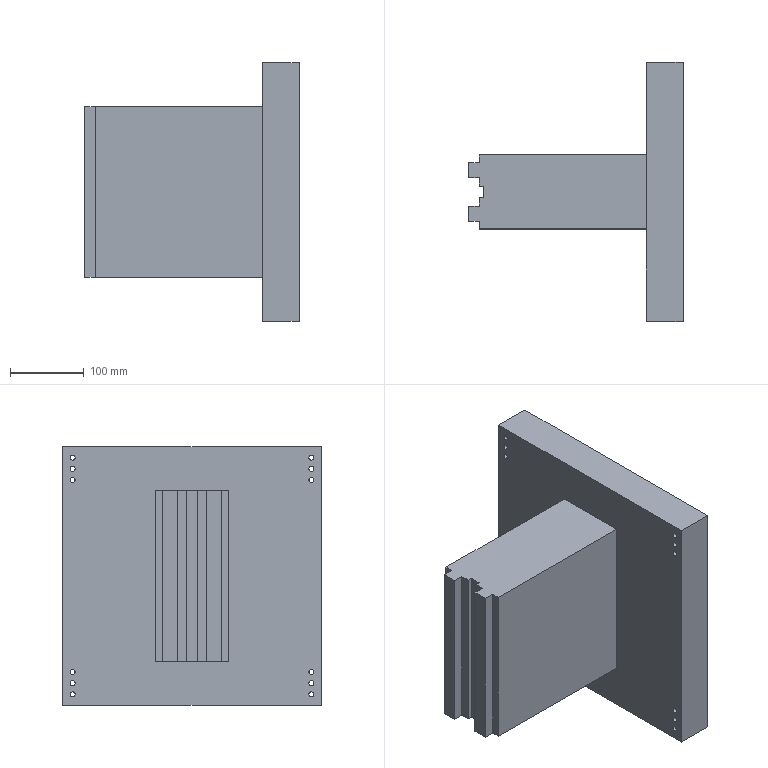Component | SolidWorks | Part8-1 | 1 solid | 47 faces | box 290 x 350 x 350 mm | volume 11409352 mm3 | cylinder 24 | plane 23 | commonest cylinder face diameters 6.793 x24
build123d program:
from build123d import *

# Parameters (mm, degrees)
SKETCH1_W           = 350
SKETCH1_H           = 350
SKETCH1_R           = 3.397
BOSS_EXTRUDE1_DEPTH = 50
SKETCH2_W           = 230
SKETCH2_H           = 100
BOSS_EXTRUDE2_DEPTH = 220
SKETCH3_W           = 230
SKETCH3_H           = 42.5
BOSS_EXTRUDE3_DEPTH = 20
SKETCH6_W           = 14
SKETCH6_H           = 10.5
SKETCH6_H_2         = 12
CUT_EXTRUDE2_DEPTH  = 454.173


with BuildPart() as part:
    # Sketch1 → Boss-Extrude1 (new body)
    with BuildSketch(Plane.XY):
        with Locations((526.175, 17.784)):
            Rectangle(SKETCH1_W, SKETCH1_H)
        with Locations((366.175, 179.28)):
            Circle(SKETCH1_R, mode=Mode.SUBTRACT)
        with Locations((381.175, 179.28)):
            Circle(SKETCH1_R, mode=Mode.SUBTRACT)
        with Locations((396.175, 179.28)):
            Circle(SKETCH1_R, mode=Mode.SUBTRACT)
        with Locations(Location((656.175, 179.28, 0), (0, 0, 180))):
            Circle(SKETCH1_R, mode=Mode.SUBTRACT)
        with Locations(Location((671.175, 179.28, 0), (0, 0, 180))):
            Circle(SKETCH1_R, mode=Mode.SUBTRACT)
        with Locations(Location((686.175, 179.28, 0), (0, 0, 180))):
            Circle(SKETCH1_R, mode=Mode.SUBTRACT)
        with Locations((686.175, -143.712)):
            Circle(SKETCH1_R, mode=Mode.SUBTRACT)
        with Locations((671.175, -143.712)):
            Circle(SKETCH1_R, mode=Mode.SUBTRACT)
        with Locations((656.175, -143.712)):
            Circle(SKETCH1_R, mode=Mode.SUBTRACT)
        with Locations(Location((396.175, -143.712, 0), (0, 0, 180))):
            Circle(SKETCH1_R, mode=Mode.SUBTRACT)
        with Locations(Location((381.175, -143.712, 0), (0, 0, 180))):
            Circle(SKETCH1_R, mode=Mode.SUBTRACT)
        with Locations(Location((366.175, -143.712, 0), (0, 0, 180))):
            Circle(SKETCH1_R, mode=Mode.SUBTRACT)
    extrude(amount=BOSS_EXTRUDE1_DEPTH)

    # Sketch2 → Boss-Extrude2 (add)
    with BuildSketch(Plane.XY.offset(50)):
        with Locations((526.175, 17.784)):
            Rectangle(SKETCH2_W, SKETCH2_H)
    extrude(amount=BOSS_EXTRUDE2_DEPTH)

    # Sketch3 → Boss-Extrude3 (add)
    with BuildSketch(Plane.XY.offset(270)):
        with Locations((526.175, -10.966)):
            Rectangle(SKETCH3_W, SKETCH3_H)
        with Locations((526.175, 46.534)):
            Rectangle(SKETCH3_W, SKETCH3_H)
    extrude(amount=BOSS_EXTRUDE3_DEPTH)

    # Sketch6 → Cut-Extrude2 (cut, through all)
    with BuildSketch(Plane.ZY.offset(-411.175)):
        with Locations((283, 62.534)):
            Rectangle(SKETCH6_W, SKETCH6_H)
        with Locations((283, 31.284)):
            Rectangle(SKETCH6_W, SKETCH6_H_2)
        with Locations((283, 4.284)):
            Rectangle(SKETCH6_W, SKETCH6_H_2)
        with Locations((283, -26.966)):
            Rectangle(SKETCH6_W, SKETCH6_H)
    extrude(amount=-CUT_EXTRUDE2_DEPTH, mode=Mode.SUBTRACT)


solid = part.part

# Placed as in the assembly
solid = solid.moved(Location((139.443, -11.952, -528.526), (0, -90, 0)))